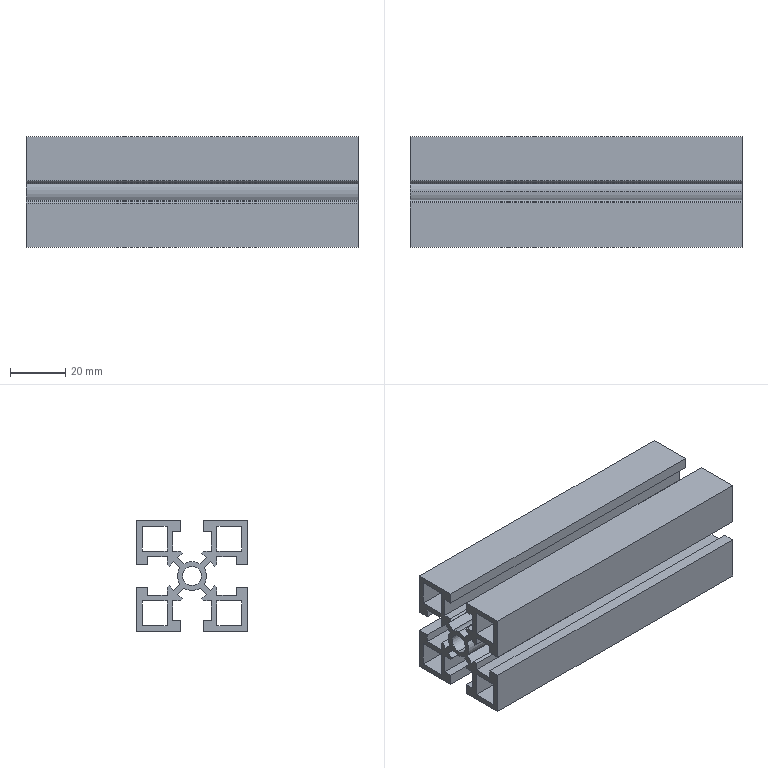Component | SolidWorks | AluminumProfile120-1 | 1 solid | 89 faces | box 120 x 40 x 40 mm | volume 69609 mm3 | plane 82 | cylinder 7 | commonest cylinder face diameters 10.5 x5 6.8 x2 | material 6061 Alloy
build123d program:
from build123d import *

# Parameters (mm, degrees)
SKETCH1_W                  = 40
SKETCH1_H                  = 40
EXTRUDE1_DEPTH             = 1640
CUT_EXTRUDE1_DEPTH         = 1641.975
SKETCH3_R                  = 3.4
CUT_EXTRUDE2_DEPTH         = 1641.975
CIRPATTERN1_COUNT          = 4
EXTRUDE2_DEPTH             = 1641.975
CIRPATTERN2_COUNT          = 4
SKETCH5_W                  = 9
SKETCH5_H                  = 9
EXTRUDE3_DEPTH             = 1641.975
CIRPATTERN3_COUNT          = 4
M8X1_25_TAPPED_HOLE3_D     = 6.8
M8X1_25_TAPPED_HOLE3_DEPTH = 19.75
M8X1_25_TAPPED_HOLE3_TIP   = 2.043
SKETCH9_W                  = 177.591
SKETCH9_H                  = 2021.808
CUT_EXTRUDE3_DEPTH         = 1641.975


with BuildPart() as part:
    # Sketch1 → Extrude1 (new body)
    with BuildSketch(Plane.XY):
        with Locations((20, 20)):
            Rectangle(SKETCH1_W, SKETCH1_H)
    extrude(amount=EXTRUDE1_DEPTH)

    # Sketch2 → Cut-Extrude1 (cut, through all)
    with BuildSketch(Plane.XY.offset(1640)):
        Polygon((16, 40), (16, 36), (13, 36), (13, 29), (27, 29), (27, 36), (24, 36), (24, 40), align=None)
    cut_extrude1 = extrude(amount=-CUT_EXTRUDE1_DEPTH, mode=Mode.SUBTRACT)

    # Sketch3 → Cut-Extrude2 (cut, through all)
    with BuildSketch(Plane.XY.offset(1640)):
        with Locations((20, 20)):
            Circle(SKETCH3_R)
    extrude(amount=-CUT_EXTRUDE2_DEPTH, mode=Mode.SUBTRACT)

    # CirPattern1: Cut-Extrude1 ×4 about axis
    cirpattern1_axis = Axis((20, 20, 0), (0, 0, 1))
    for i in range(1, CIRPATTERN1_COUNT):
        add(cut_extrude1.rotate(cirpattern1_axis, i * 360 / CIRPATTERN1_COUNT), mode=Mode.SUBTRACT)

    # Sketch4 → Extrude2 (cut, through all)
    with BuildSketch(Plane.XY.offset(1640)):
        with BuildLine():
            Line((15.75, 29), (16.457, 28.293))
            Line((16.457, 28.293), (14.806, 26.641))
            Line((14.806, 26.641), (17.082, 24.365))
            ThreePointArc((17.082, 24.365), (20, 25.25), (22.918, 24.365))
            Line((22.918, 24.365), (25.194, 26.641))
            Line((25.194, 26.641), (23.543, 28.293))
            Line((23.543, 28.293), (24.25, 29))
            Line((24.25, 29), (15.75, 29))
        make_face()
    extrude2 = extrude(amount=-EXTRUDE2_DEPTH, mode=Mode.SUBTRACT)

    # CirPattern2: Extrude2 ×4 about axis
    cirpattern2_axis = Axis((20, 20, 0), (0, 0, 1))
    for i in range(1, CIRPATTERN2_COUNT):
        add(extrude2.rotate(cirpattern2_axis, i * 360 / CIRPATTERN2_COUNT), mode=Mode.SUBTRACT)

    # Sketch5 → Extrude3 (cut, through all)
    with BuildSketch(Plane.XY.offset(1640)):
        with Locations((6.5, 33.5)):
            Rectangle(SKETCH5_W, SKETCH5_H)
    extrude3 = extrude(amount=-EXTRUDE3_DEPTH, mode=Mode.SUBTRACT)

    # CirPattern3: Extrude3 ×4 about axis
    cirpattern3_axis = Axis((20, 20, 0), (0, 0, 1))
    for i in range(1, CIRPATTERN3_COUNT):
        add(extrude3.rotate(cirpattern3_axis, i * 360 / CIRPATTERN3_COUNT), mode=Mode.SUBTRACT)

    # M8x1.25 Tapped Hole3
    with Locations(Plane(origin=(20, 20, 1640), x_dir=(1, 0, 0), z_dir=(0, 0, 1))):
        with Locations((0, 0)):
            Hole(M8X1_25_TAPPED_HOLE3_D / 2, depth=M8X1_25_TAPPED_HOLE3_DEPTH)
            with Locations((0, 0, -(M8X1_25_TAPPED_HOLE3_DEPTH + M8X1_25_TAPPED_HOLE3_TIP / 2))):  # 118° drill point
                Cone(0, M8X1_25_TAPPED_HOLE3_D / 2, M8X1_25_TAPPED_HOLE3_TIP, mode=Mode.SUBTRACT)

    # Sketch9 → Cut-Extrude3 (cut, through all)
    with BuildSketch(Plane.XZ):
        with Locations((13.869, 1130.904)):
            Rectangle(SKETCH9_W, SKETCH9_H)
    extrude(amount=-CUT_EXTRUDE3_DEPTH, mode=Mode.SUBTRACT)


solid = part.part

# Placed as in the assembly
solid = solid.moved(Location((-888.352, 51.783, 683.715), (0, 90, 0)))